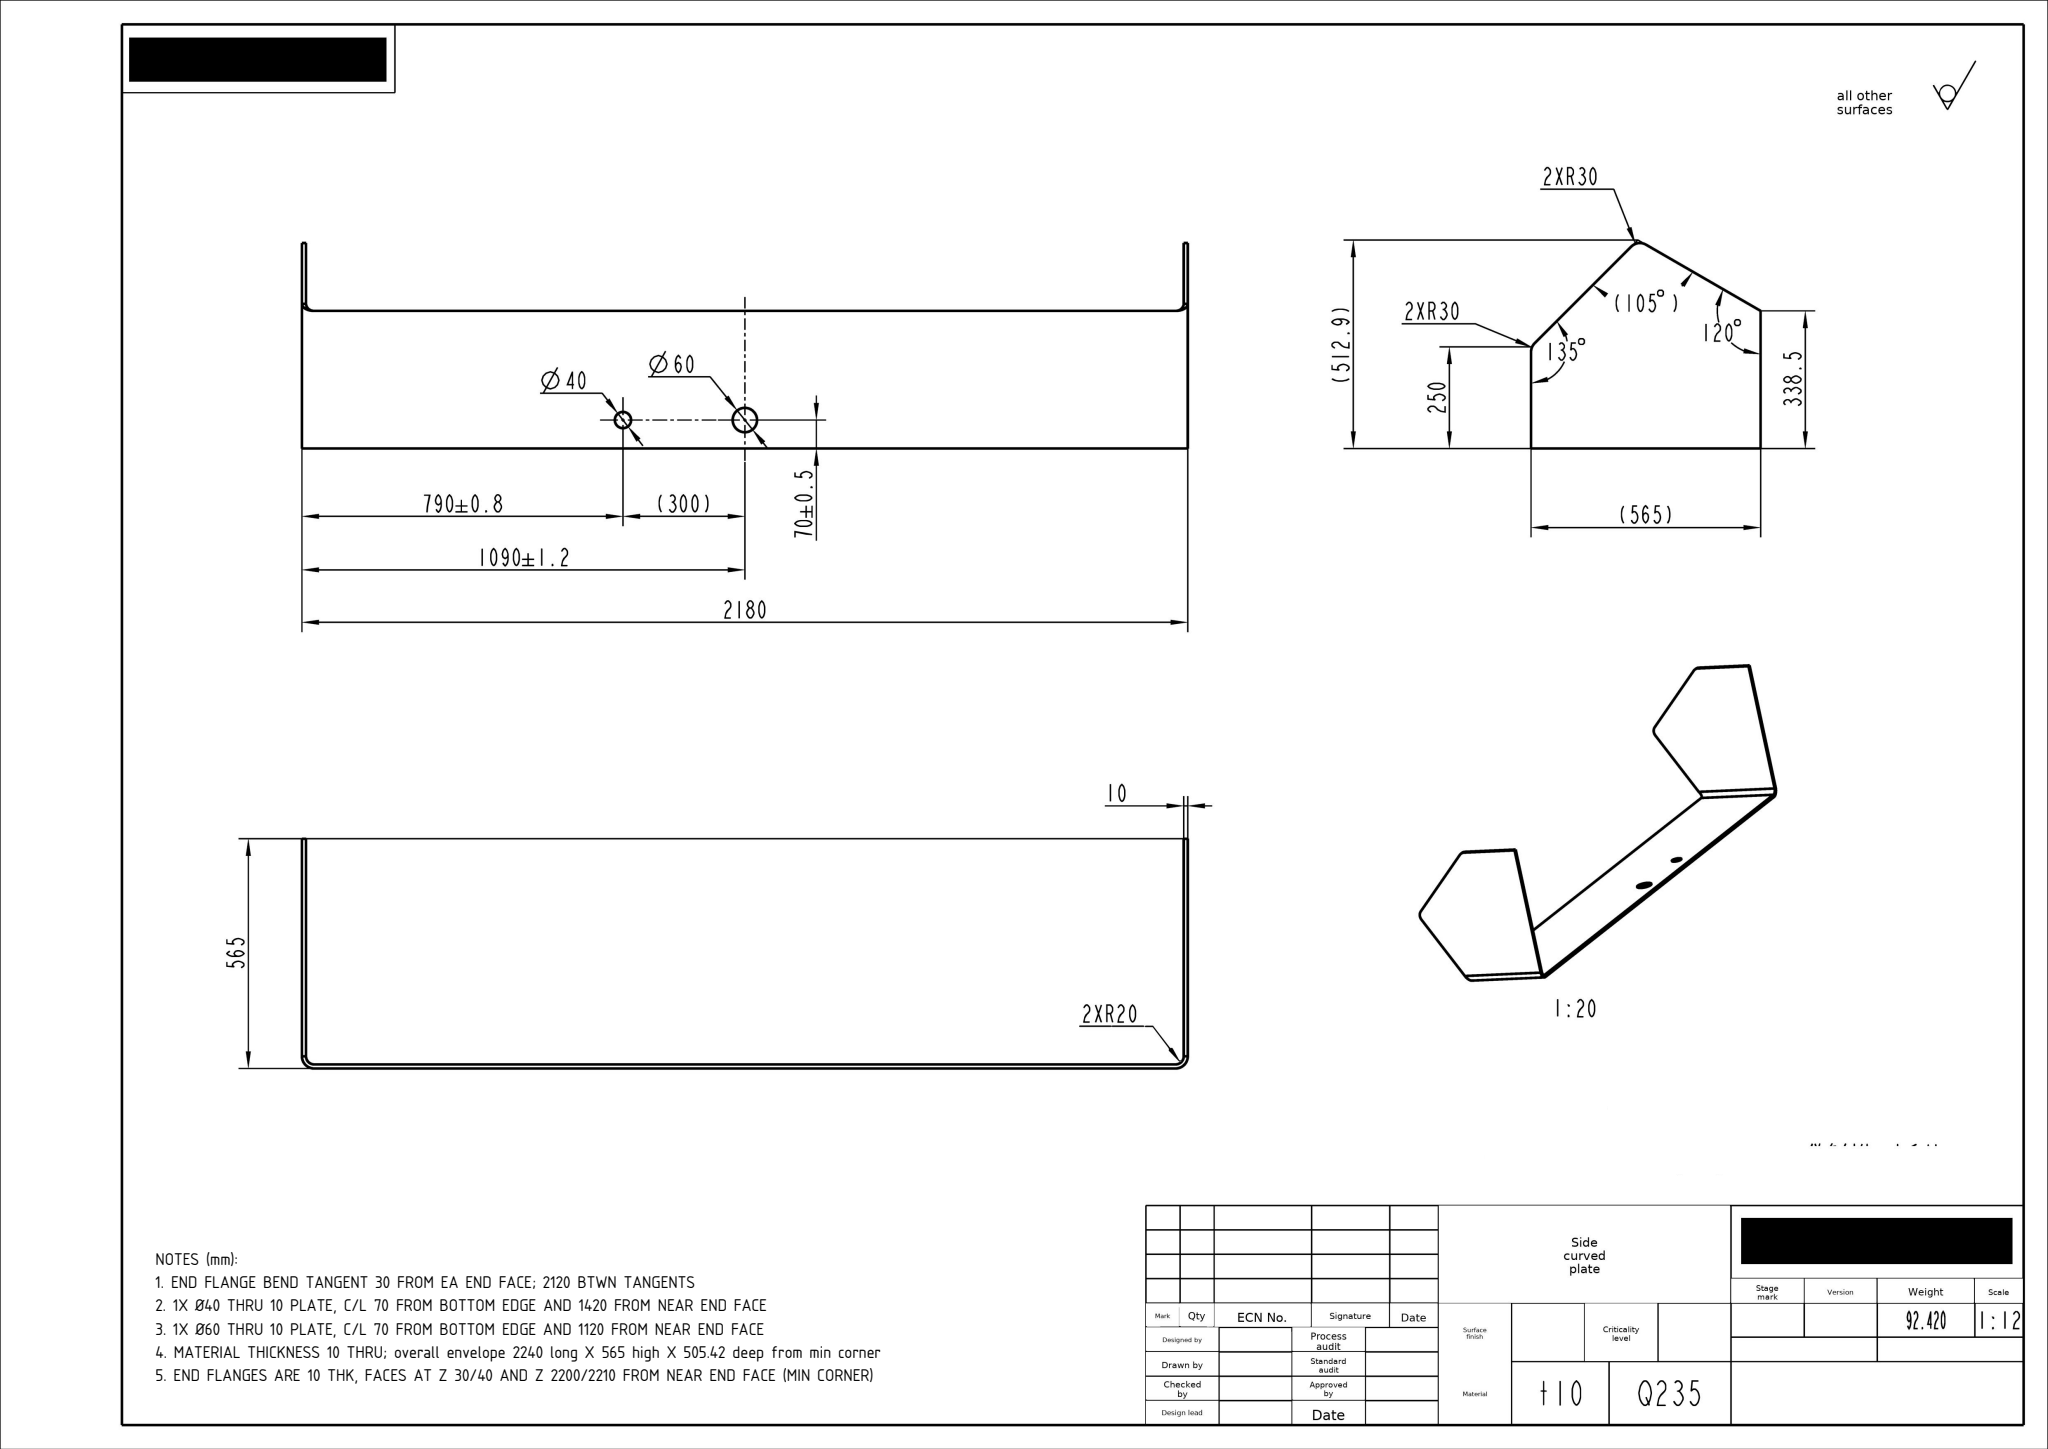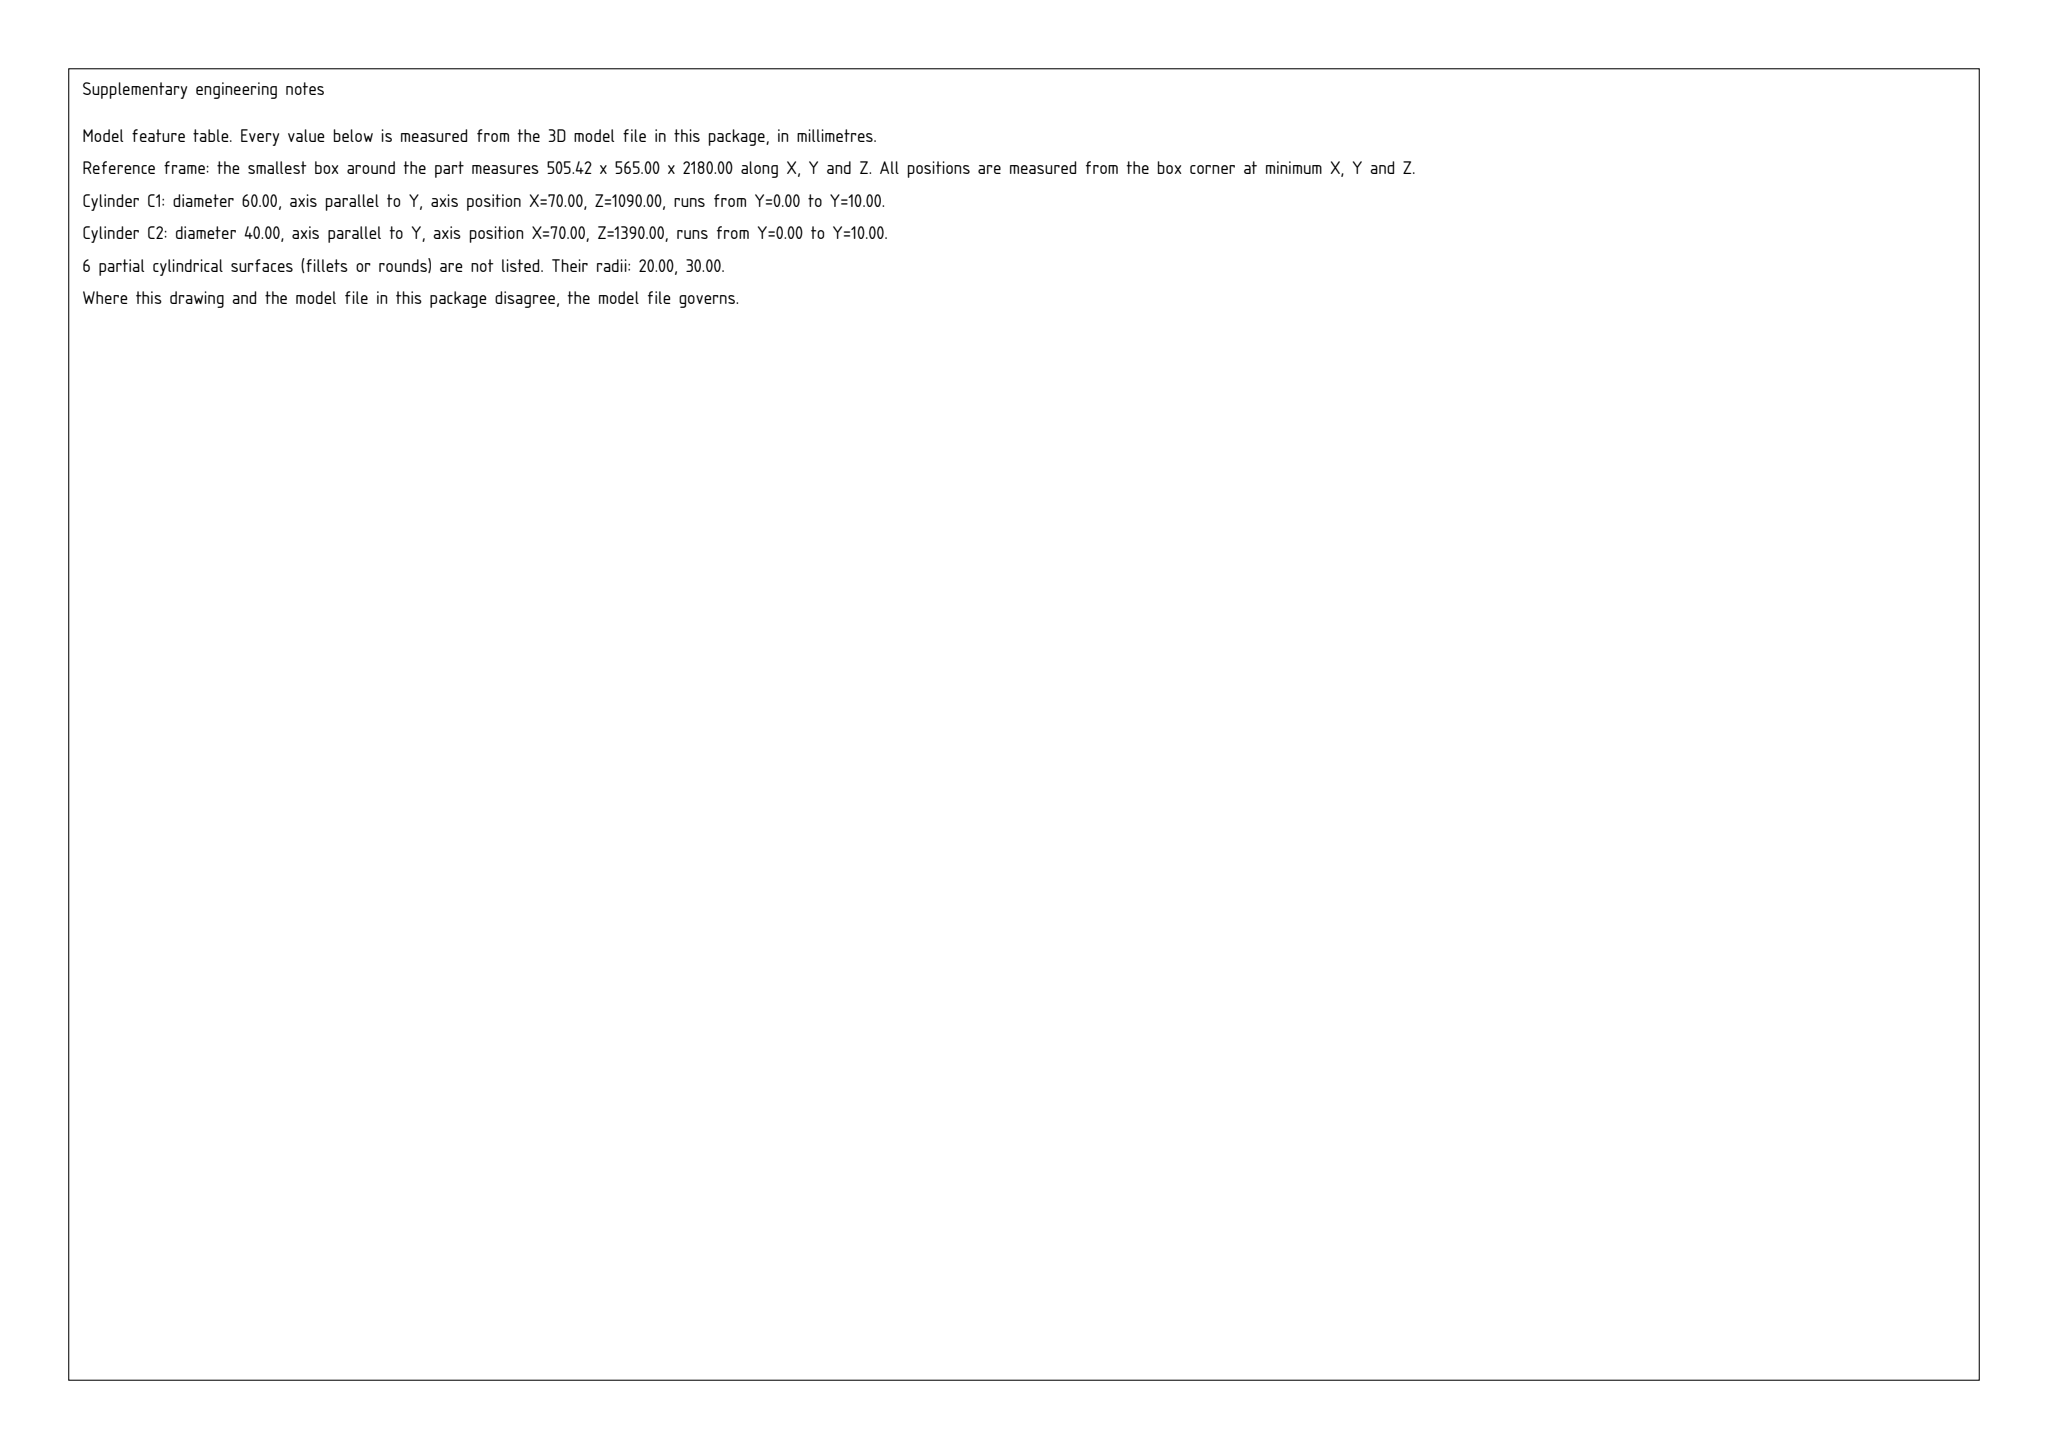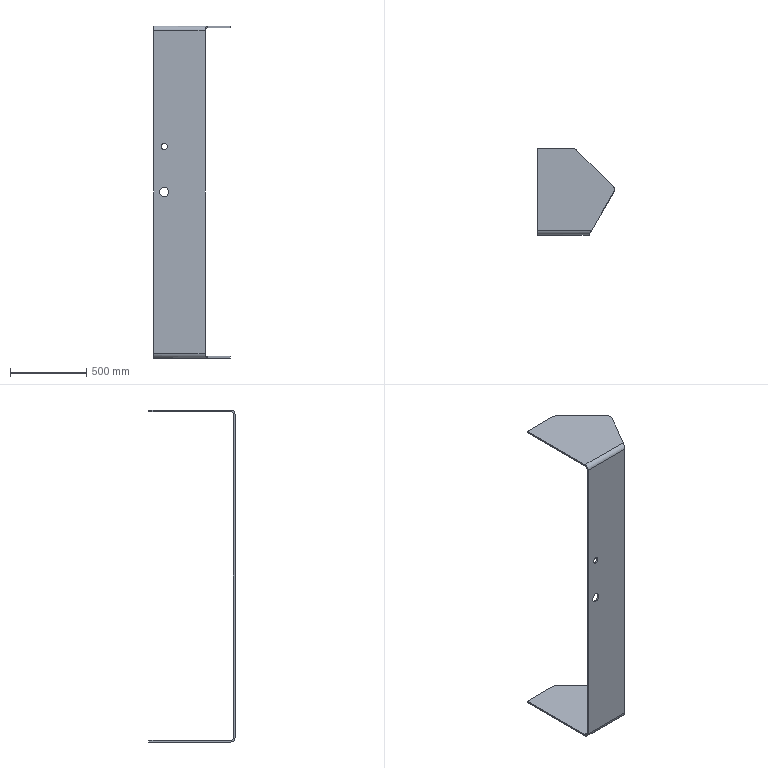Part | SolidWorks | mm | 1 solid | 33 faces | box 505.42 x 565 x 2180 mm | volume 11773242 mm3 | plane 18 | cylinder 13 | spline 2 | commonest cylinder face diameters 60 x9 40 x4
Drawing notes:
END FLANGE BEND TANGENT 30 FROM EA END FACE; 2120 BTWN TANGENTS | from the solid: Bend fillet cyls axis x at z=60 and z=2180 (R20 inner/R30 outer, ctr y=30); end faces at z=30 and z=2210 (2180 OAL); 2180-2x30=2120
1X Ø40 THRU 10 PLATE, C/L 70 FROM BOTTOM EDGE AND 1420 FROM NEAR END FACE | from the solid: cylinders [40.0,"y",[70.0,null,1420.0],10.0]
1X Ø60 THRU 10 PLATE, C/L 70 FROM BOTTOM EDGE AND 1120 FROM NEAR END FACE | from the solid: cylinders [60.0,"y",[70.0,null,1120.0],10.0]
MATERIAL THICKNESS 10 THRU; overall envelope 2240 long X 565 high X 505.42 deep from min corner | from the solid: bbox_xyz [505.42, 565.0, 2240.0]; axis_planes y=0.0 and y=10.0
END FLANGES ARE 10 THK, FACES AT Z 30/40 AND Z 2200/2210 FROM NEAR END FACE (MIN CORNER) | from the solid: axis_planes ["z",30.0],["z",40.0],["z",2200.0],["z",2210.0]